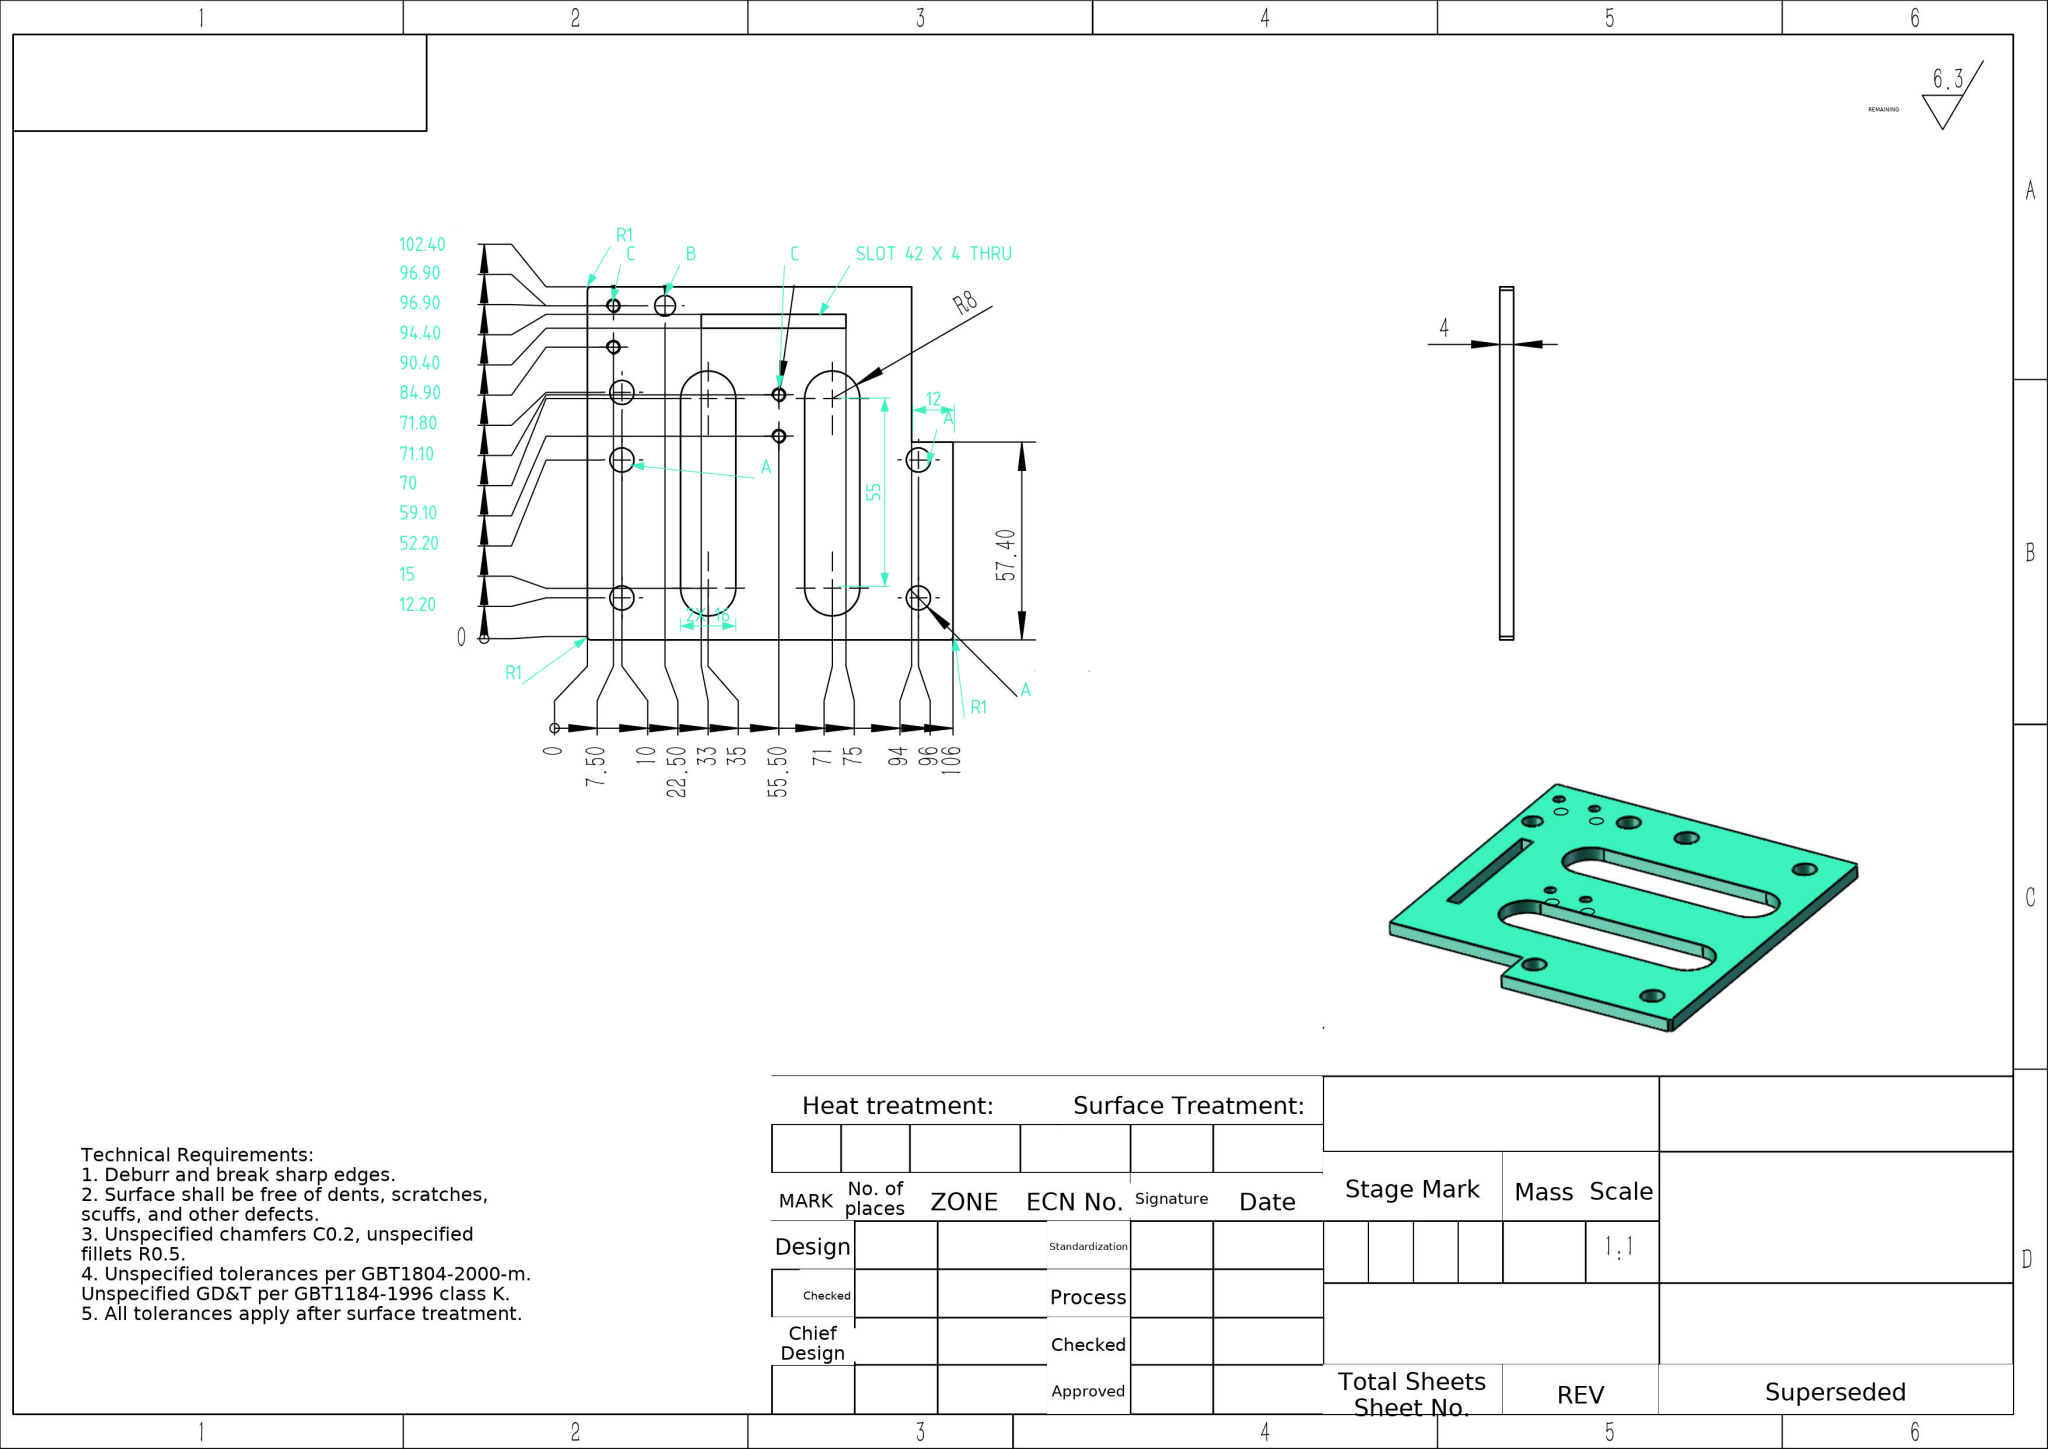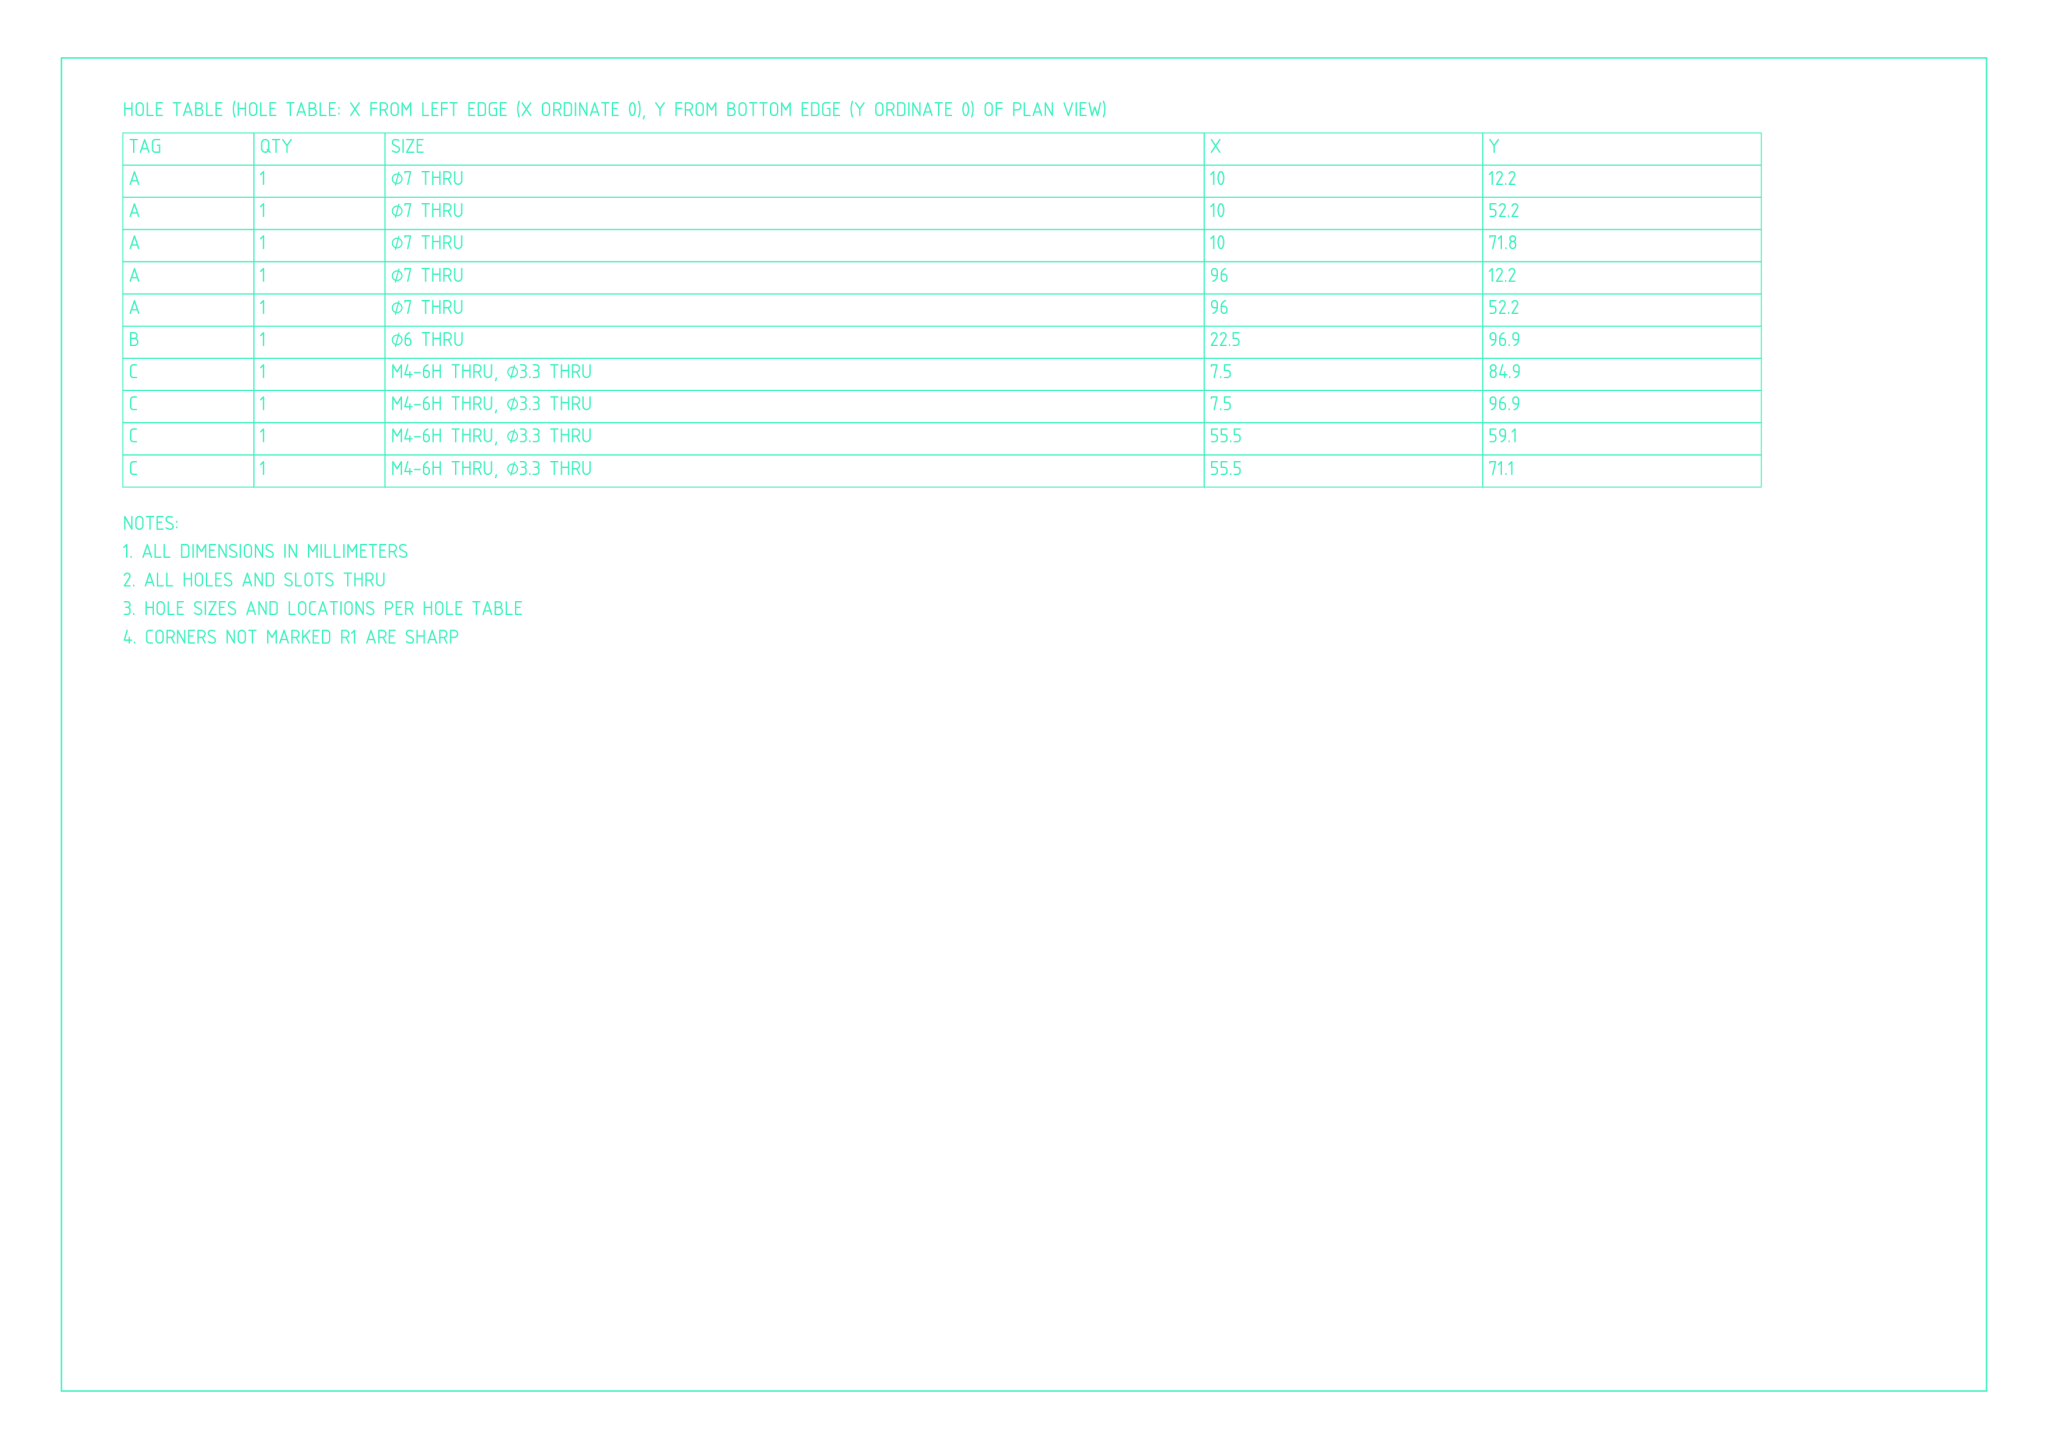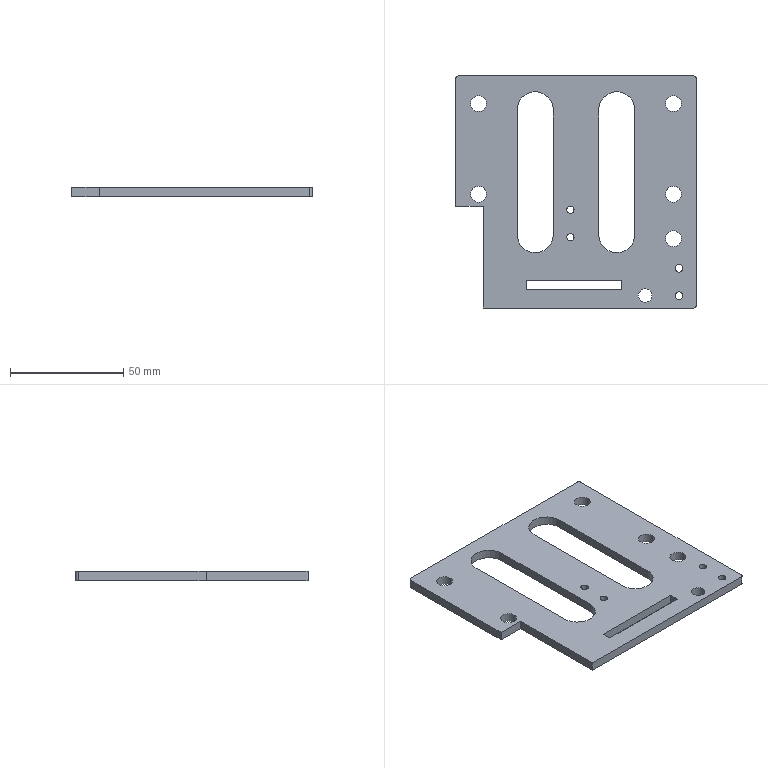Part | NX | mm | 1 solid | 43 faces | box 106 x 102.4 x 4 mm | volume 30915 mm3 | cylinder 27 | plane 16 | commonest cylinder face diameters 7 x10 3.3 x8 16 x4 2 x3 6 x2